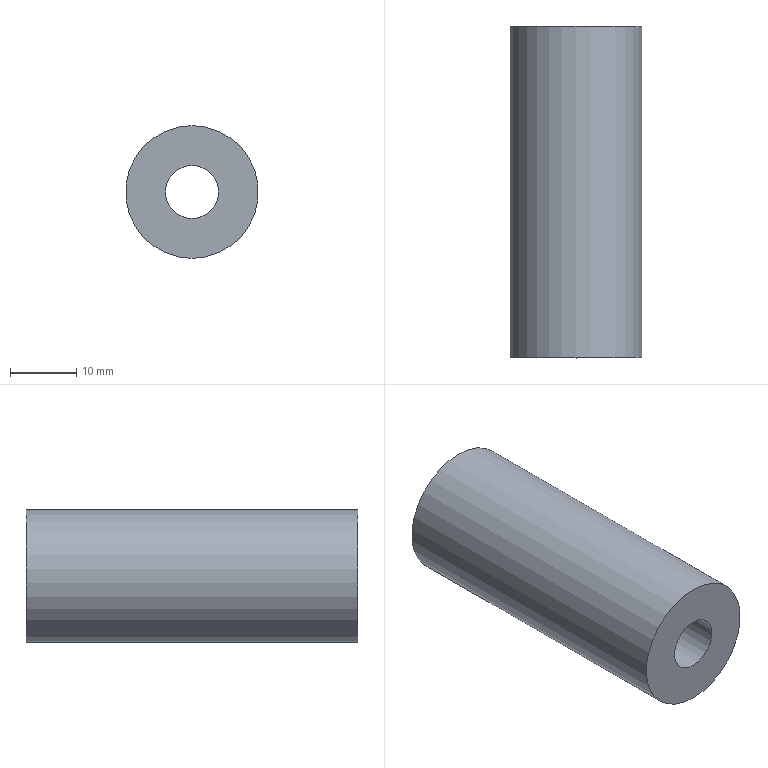Component | NX | COUPLING_2 | 1 solid | 4 faces | box 20 x 50 x 20 mm | volume 13195 mm3 | cylinder 2 | plane 2 | commonest cylinder face diameters 20 x1 8 x1
STEP:
#1=CARTESIAN_POINT('',(0.,0.,0.));
#2=DIRECTION('',(0.,0.,1.));
#3=DIRECTION('',(1.,0.,0.));
#4=AXIS2_PLACEMENT_3D('',#1,#2,#3);
#5=CARTESIAN_POINT('',(630.189,-369.302,-1486.));
#6=VERTEX_POINT('',#5);
#7=CARTESIAN_POINT('',(630.189,-369.302,-1476.));
#8=DIRECTION('',(0.,-1.,0.));
#9=DIRECTION('',(0.,0.,-1.));
#10=AXIS2_PLACEMENT_3D('',#7,#8,#9);
#11=CIRCLE('',#10,10.);
#12=CARTESIAN_POINT('',(630.189,-369.302,-1476.));
#13=DIRECTION('',(0.,1.,0.));
#14=DIRECTION('',(0.,0.,1.));
#15=AXIS2_PLACEMENT_3D('',#12,#13,#14);
#16=CYLINDRICAL_SURFACE('',#15,10.);
#17=CARTESIAN_POINT('',(9.425,0.));
#18=DIRECTION('',(-1.,0.));
#19=VECTOR('',#18,1.);
#20=LINE('',#17,#19);
#21=(GEOMETRIC_REPRESENTATION_CONTEXT(2)PARAMETRIC_REPRESENTATION_CONTEXT()REPRESENTATION_CONTEXT('',''));
#22=DEFINITIONAL_REPRESENTATION('',(#20),#21);
#23=PCURVE('',#16,#22);
#24=CARTESIAN_POINT('',(630.189,-369.302,-1476.));
#25=DIRECTION('',(0.,-1.,0.));
#26=DIRECTION('',(0.,0.,-1.));
#27=AXIS2_PLACEMENT_3D('',#24,#25,#26);
#28=PLANE('',#27);
#29=CARTESIAN_POINT('',(0.,0.));
#30=DIRECTION('',(1.,0.));
#31=AXIS2_PLACEMENT_2D('',#29,#30);
#32=CIRCLE('',#31,10.);
#33=(GEOMETRIC_REPRESENTATION_CONTEXT(2)PARAMETRIC_REPRESENTATION_CONTEXT()REPRESENTATION_CONTEXT('',''));
#34=DEFINITIONAL_REPRESENTATION('',(#32),#33);
#35=PCURVE('',#28,#34);
#36=SURFACE_CURVE('',#11,(#23,#35),.PCURVE_S1.);
#37=EDGE_CURVE('',#6,#6,#36,.T.);
#38=ORIENTED_EDGE('',*,*,#37,.F.);
#39=CARTESIAN_POINT('',(630.189,-319.302,-1486.));
#40=VERTEX_POINT('',#39);
#41=CARTESIAN_POINT('',(630.189,-369.302,-1486.));
#42=CARTESIAN_POINT('',(630.189,-319.302,-1486.));
#43=B_SPLINE_CURVE_WITH_KNOTS('',1,(#41,#42),.UNSPECIFIED.,.F.,.F.,(2,2),(0.,50.),.PIECEWISE_BEZIER_KNOTS.);
#44=CARTESIAN_POINT('',(9.425,0.));
#45=DIRECTION('',(0.,1.));
#46=VECTOR('',#45,1.);
#47=LINE('',#44,#46);
#48=(GEOMETRIC_REPRESENTATION_CONTEXT(2)PARAMETRIC_REPRESENTATION_CONTEXT()REPRESENTATION_CONTEXT('',''));
#49=DEFINITIONAL_REPRESENTATION('',(#47),#48);
#50=PCURVE('',#16,#49);
#51=CARTESIAN_POINT('',(3.142,0.));
#52=DIRECTION('',(0.,1.));
#53=VECTOR('',#52,1.);
#54=LINE('',#51,#53);
#55=(GEOMETRIC_REPRESENTATION_CONTEXT(2)PARAMETRIC_REPRESENTATION_CONTEXT()REPRESENTATION_CONTEXT('',''));
#56=DEFINITIONAL_REPRESENTATION('',(#54),#55);
#57=PCURVE('',#16,#56);
#58=SEAM_CURVE('',#43,(#50,#57),.PCURVE_S1.);
#59=EDGE_CURVE('',#6,#40,#58,.T.);
#60=ORIENTED_EDGE('',*,*,#59,.T.);
#61=CARTESIAN_POINT('',(630.189,-319.302,-1476.));
#62=DIRECTION('',(0.,-1.,0.));
#63=DIRECTION('',(0.,0.,-1.));
#64=AXIS2_PLACEMENT_3D('',#61,#62,#63);
#65=CIRCLE('',#64,10.);
#66=CARTESIAN_POINT('',(9.425,50.));
#67=DIRECTION('',(-1.,0.));
#68=VECTOR('',#67,1.);
#69=LINE('',#66,#68);
#70=(GEOMETRIC_REPRESENTATION_CONTEXT(2)PARAMETRIC_REPRESENTATION_CONTEXT()REPRESENTATION_CONTEXT('',''));
#71=DEFINITIONAL_REPRESENTATION('',(#69),#70);
#72=PCURVE('',#16,#71);
#73=CARTESIAN_POINT('',(630.189,-319.302,-1476.));
#74=DIRECTION('',(0.,-1.,0.));
#75=DIRECTION('',(0.,0.,-1.));
#76=AXIS2_PLACEMENT_3D('',#73,#74,#75);
#77=PLANE('',#76);
#78=CARTESIAN_POINT('',(0.,0.));
#79=DIRECTION('',(1.,0.));
#80=AXIS2_PLACEMENT_2D('',#78,#79);
#81=CIRCLE('',#80,10.);
#82=(GEOMETRIC_REPRESENTATION_CONTEXT(2)PARAMETRIC_REPRESENTATION_CONTEXT()REPRESENTATION_CONTEXT('',''));
#83=DEFINITIONAL_REPRESENTATION('',(#81),#82);
#84=PCURVE('',#77,#83);
#85=SURFACE_CURVE('',#65,(#72,#84),.PCURVE_S1.);
#86=EDGE_CURVE('',#40,#40,#85,.T.);
#87=ORIENTED_EDGE('',*,*,#86,.T.);
#88=ORIENTED_EDGE('',*,*,#59,.F.);
#89=EDGE_LOOP('',(#38,#60,#87,#88));
#90=FACE_BOUND('',#89,.T.);
#91=ADVANCED_FACE('',(#90),#16,.T.);
#92=CARTESIAN_POINT('',(630.189,-369.302,-1480.));
#93=VERTEX_POINT('',#92);
#94=CARTESIAN_POINT('',(630.189,-369.302,-1476.));
#95=DIRECTION('',(0.,-1.,0.));
#96=DIRECTION('',(0.,0.,-1.));
#97=AXIS2_PLACEMENT_3D('',#94,#95,#96);
#98=CIRCLE('',#97,4.);
#99=CARTESIAN_POINT('',(630.189,-369.302,-1476.));
#100=DIRECTION('',(0.,1.,0.));
#101=DIRECTION('',(0.,0.,1.));
#102=AXIS2_PLACEMENT_3D('',#99,#100,#101);
#103=CYLINDRICAL_SURFACE('',#102,4.);
#104=CARTESIAN_POINT('',(9.425,0.));
#105=DIRECTION('',(-1.,0.));
#106=VECTOR('',#105,1.);
#107=LINE('',#104,#106);
#108=(GEOMETRIC_REPRESENTATION_CONTEXT(2)PARAMETRIC_REPRESENTATION_CONTEXT()REPRESENTATION_CONTEXT('',''));
#109=DEFINITIONAL_REPRESENTATION('',(#107),#108);
#110=PCURVE('',#103,#109);
#111=CARTESIAN_POINT('',(0.,0.));
#112=DIRECTION('',(1.,0.));
#113=AXIS2_PLACEMENT_2D('',#111,#112);
#114=CIRCLE('',#113,4.);
#115=(GEOMETRIC_REPRESENTATION_CONTEXT(2)PARAMETRIC_REPRESENTATION_CONTEXT()REPRESENTATION_CONTEXT('',''));
#116=DEFINITIONAL_REPRESENTATION('',(#114),#115);
#117=PCURVE('',#28,#116);
#118=SURFACE_CURVE('',#98,(#110,#117),.PCURVE_S1.);
#119=EDGE_CURVE('',#93,#93,#118,.T.);
#120=ORIENTED_EDGE('',*,*,#119,.F.);
#121=CARTESIAN_POINT('',(630.189,-319.302,-1480.));
#122=VERTEX_POINT('',#121);
#123=CARTESIAN_POINT('',(630.189,-369.302,-1480.));
#124=CARTESIAN_POINT('',(630.189,-319.302,-1480.));
#125=B_SPLINE_CURVE_WITH_KNOTS('',1,(#123,#124),.UNSPECIFIED.,.F.,.F.,(2,2),(0.,50.),.PIECEWISE_BEZIER_KNOTS.);
#126=CARTESIAN_POINT('',(9.425,0.));
#127=DIRECTION('',(0.,1.));
#128=VECTOR('',#127,1.);
#129=LINE('',#126,#128);
#130=(GEOMETRIC_REPRESENTATION_CONTEXT(2)PARAMETRIC_REPRESENTATION_CONTEXT()REPRESENTATION_CONTEXT('',''));
#131=DEFINITIONAL_REPRESENTATION('',(#129),#130);
#132=PCURVE('',#103,#131);
#133=CARTESIAN_POINT('',(3.142,0.));
#134=DIRECTION('',(0.,1.));
#135=VECTOR('',#134,1.);
#136=LINE('',#133,#135);
#137=(GEOMETRIC_REPRESENTATION_CONTEXT(2)PARAMETRIC_REPRESENTATION_CONTEXT()REPRESENTATION_CONTEXT('',''));
#138=DEFINITIONAL_REPRESENTATION('',(#136),#137);
#139=PCURVE('',#103,#138);
#140=SEAM_CURVE('',#125,(#132,#139),.PCURVE_S1.);
#141=EDGE_CURVE('',#93,#122,#140,.T.);
#142=ORIENTED_EDGE('',*,*,#141,.T.);
#143=CARTESIAN_POINT('',(630.189,-319.302,-1476.));
#144=DIRECTION('',(0.,-1.,0.));
#145=DIRECTION('',(0.,0.,-1.));
#146=AXIS2_PLACEMENT_3D('',#143,#144,#145);
#147=CIRCLE('',#146,4.);
#148=CARTESIAN_POINT('',(9.425,50.));
#149=DIRECTION('',(-1.,0.));
#150=VECTOR('',#149,1.);
#151=LINE('',#148,#150);
#152=(GEOMETRIC_REPRESENTATION_CONTEXT(2)PARAMETRIC_REPRESENTATION_CONTEXT()REPRESENTATION_CONTEXT('',''));
#153=DEFINITIONAL_REPRESENTATION('',(#151),#152);
#154=PCURVE('',#103,#153);
#155=CARTESIAN_POINT('',(0.,0.));
#156=DIRECTION('',(1.,0.));
#157=AXIS2_PLACEMENT_2D('',#155,#156);
#158=CIRCLE('',#157,4.);
#159=(GEOMETRIC_REPRESENTATION_CONTEXT(2)PARAMETRIC_REPRESENTATION_CONTEXT()REPRESENTATION_CONTEXT('',''));
#160=DEFINITIONAL_REPRESENTATION('',(#158),#159);
#161=PCURVE('',#77,#160);
#162=SURFACE_CURVE('',#147,(#154,#161),.PCURVE_S1.);
#163=EDGE_CURVE('',#122,#122,#162,.T.);
#164=ORIENTED_EDGE('',*,*,#163,.T.);
#165=ORIENTED_EDGE('',*,*,#141,.F.);
#166=EDGE_LOOP('',(#120,#142,#164,#165));
#167=FACE_BOUND('',#166,.F.);
#168=ADVANCED_FACE('',(#167),#103,.F.);
#169=ORIENTED_EDGE('',*,*,#37,.T.);
#170=EDGE_LOOP('',(#169));
#171=FACE_BOUND('',#170,.T.);
#172=ORIENTED_EDGE('',*,*,#119,.F.);
#173=EDGE_LOOP('',(#172));
#174=FACE_BOUND('',#173,.T.);
#175=ADVANCED_FACE('',(#171,#174),#28,.T.);
#176=ORIENTED_EDGE('',*,*,#86,.F.);
#177=EDGE_LOOP('',(#176));
#178=FACE_BOUND('',#177,.T.);
#179=ORIENTED_EDGE('',*,*,#163,.T.);
#180=EDGE_LOOP('',(#179));
#181=FACE_BOUND('',#180,.T.);
#182=ADVANCED_FACE('',(#178,#181),#77,.F.);
#183=CLOSED_SHELL('',(#91,#168,#175,#182));
#184=MANIFOLD_SOLID_BREP('',#183);
#185=(LENGTH_UNIT()NAMED_UNIT(*)SI_UNIT(.MILLI.,.METRE.));
#186=UNCERTAINTY_MEASURE_WITH_UNIT(LENGTH_MEASURE(0.00001),#185,'','');
#187=(NAMED_UNIT(*)PLANE_ANGLE_UNIT()SI_UNIT($,.RADIAN.));
#188=(NAMED_UNIT(*)SI_UNIT($,.STERADIAN.)SOLID_ANGLE_UNIT());
#189=(GEOMETRIC_REPRESENTATION_CONTEXT(3)GLOBAL_UNCERTAINTY_ASSIGNED_CONTEXT((#186))GLOBAL_UNIT_ASSIGNED_CONTEXT((#185,#187,#188))REPRESENTATION_CONTEXT('',''));
#190=ADVANCED_BREP_SHAPE_REPRESENTATION('',(#4,#184),#189);